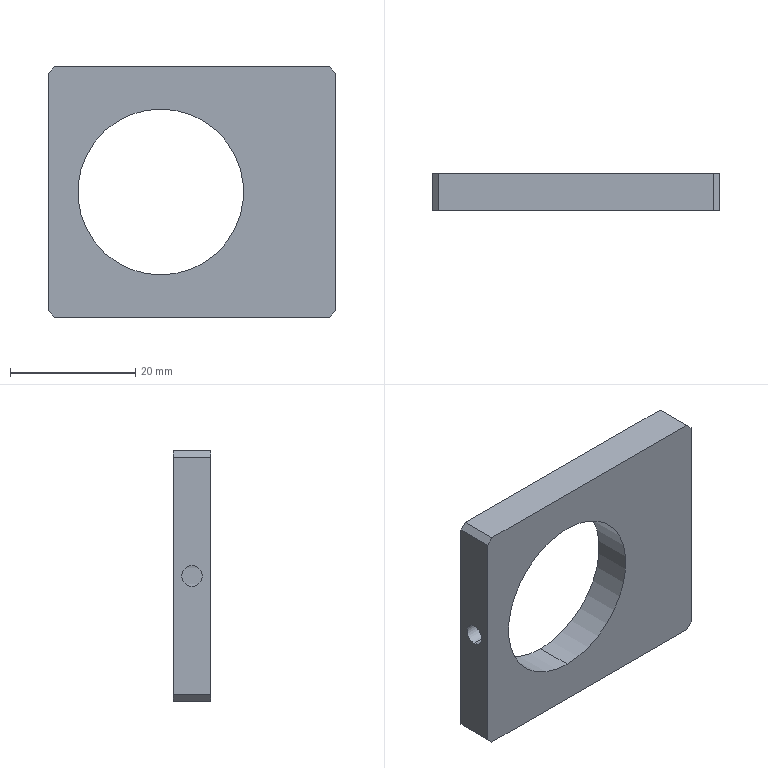Component | SolidWorks | MTCTV2104DJ006-000-0040LimitingPart-1 | 1 solid | 22 faces | box 46 x 6 x 40 mm | volume 7499 mm3 | plane 10 | cylinder 8 | cone 4 | commonest cylinder face diameters 3.3 x6 26.5 x2
build123d program:
from build123d import *

# Parameters (mm, degrees)
SKETCH1_W              = 40
SKETCH1_H              = 46
BOSS_EXTRUDE1_DEPTH    = 6
SKETCH4_R              = 13.25
CUT_EXTRUDE1_DEPTH     = 32.064
M4_TAPPED_HOLE1_REACH  = 52.517
M4_TAPPED_HOLE1_BORE_R = 1.65
M4_TAPPED_HOLE2_D      = 3.3
M4_TAPPED_HOLE2_DEPTH  = 10.1
M4_TAPPED_HOLE2_TIP    = 0.9914
CHAMFER1_SIZE          = 1


with BuildPart() as part:
    # Sketch1 → Boss-Extrude1 (new body)
    with BuildSketch(Plane(origin=(0, 0, 0), x_dir=(0, 0, -1), z_dir=(1, 0, 0))):
        Rectangle(SKETCH1_W, SKETCH1_H)
    extrude(amount=BOSS_EXTRUDE1_DEPTH)

    # Sketch4 → Cut-Extrude1 (cut, through all)
    with BuildSketch(Plane(origin=(6, 0, 0), x_dir=(0, 0, -1), z_dir=(1, 0, 0))):
        with Locations((0, -5)):
            Circle(SKETCH4_R)
    extrude(amount=-CUT_EXTRUDE1_DEPTH, mode=Mode.SUBTRACT)

    # M4 Tapped Hole1 bore → M4 Tapped Hole1 (cut, up to next)
    with BuildSketch(Plane(origin=(0, -23, 0), x_dir=(-1, 0, 0), z_dir=(0, -1, 0)), mode=Mode.PRIVATE) as m4_tapped_hole1_sk1:
        with Locations((-3, 0)):
            Circle(M4_TAPPED_HOLE1_BORE_R)
    m4_tapped_hole1_tool1 = extrude(m4_tapped_hole1_sk1.sketch, amount=-M4_TAPPED_HOLE1_REACH, mode=Mode.PRIVATE) & part.part
    add(m4_tapped_hole1_tool1.solids().sort_by_distance((3, -23, 0))[0], mode=Mode.SUBTRACT)

    # M4 Tapped Hole2
    with Locations(Plane(origin=(0, 23, 0), x_dir=(1, 0, 0), z_dir=(0, 1, 0))):
        with Locations((3, 16), (3, -16)):
            Hole(M4_TAPPED_HOLE2_D / 2, depth=M4_TAPPED_HOLE2_DEPTH)
            with Locations((0, 0, -(M4_TAPPED_HOLE2_DEPTH + M4_TAPPED_HOLE2_TIP / 2))):  # 118° drill point
                Cone(0, M4_TAPPED_HOLE2_D / 2, M4_TAPPED_HOLE2_TIP, mode=Mode.SUBTRACT)

    # Chamfer1
    chamfer1_edges = [part.edges().sort_by_distance(p)[0] for p in [
        (3, -23, -20),
        (3, -23, 20),
        (3, 23, 20),
        (3, 23, -20),
    ]]
    chamfer(chamfer1_edges, length=CHAMFER1_SIZE)


solid = part.part

# Placed as in the assembly
solid = solid.moved(Location((8.798, -27.678, 265.447), (0, 0, -90)))
STEP:
#1=COLOUR_RGB('',0.7922,0.8196,0.9333);
#2=FILL_AREA_STYLE_COLOUR('',#1);
#3=FILL_AREA_STYLE('',(#2));
#4=SURFACE_STYLE_FILL_AREA(#3);
#5=SURFACE_SIDE_STYLE('',(#4));
#6=SURFACE_STYLE_USAGE(.BOTH.,#5);
#7=PRESENTATION_STYLE_ASSIGNMENT((#6));
#8=CARTESIAN_POINT('',(0.8543,-1.208,11.146));
#9=VERTEX_POINT('',#8);
#10=CARTESIAN_POINT('',(0.8543,-1.208,11.016));
#11=VERTEX_POINT('',#10);
#12=CARTESIAN_POINT('',(0.8543,-1.208,11.081));
#13=DIRECTION('',(1.,0.,0.));
#14=DIRECTION('',(0.,0.,-1.));
#15=AXIS2_PLACEMENT_3D('',#12,#13,#14);
#16=CIRCLE('',#15,0.06496);
#17=EDGE_CURVE('',#9,#11,#16,.T.);
#18=ORIENTED_EDGE('',*,*,#17,.F.);
#19=CARTESIAN_POINT('',(1.252,-1.208,11.146));
#20=VERTEX_POINT('',#19);
#21=CARTESIAN_POINT('',(1.252,-1.208,11.146));
#22=DIRECTION('',(1.,0.,0.));
#23=VECTOR('',#22,39.37);
#24=LINE('',#21,#23);
#25=EDGE_CURVE('',#9,#20,#24,.T.);
#26=ORIENTED_EDGE('',*,*,#25,.T.);
#27=CARTESIAN_POINT('',(1.252,-1.208,11.016));
#28=VERTEX_POINT('',#27);
#29=CARTESIAN_POINT('',(1.252,-1.208,11.081));
#30=DIRECTION('',(1.,0.,0.));
#31=DIRECTION('',(0.,0.,-1.));
#32=AXIS2_PLACEMENT_3D('',#29,#30,#31);
#33=CIRCLE('',#32,0.06496);
#34=EDGE_CURVE('',#20,#28,#33,.T.);
#35=ORIENTED_EDGE('',*,*,#34,.T.);
#36=CARTESIAN_POINT('',(1.252,-1.208,11.016));
#37=DIRECTION('',(1.,0.,0.));
#38=VECTOR('',#37,39.37);
#39=LINE('',#36,#38);
#40=EDGE_CURVE('',#11,#28,#39,.T.);
#41=ORIENTED_EDGE('',*,*,#40,.F.);
#42=EDGE_LOOP('',(#18,#26,#35,#41));
#43=FACE_OUTER_BOUND('',#42,.T.);
#44=CARTESIAN_POINT('',(1.252,-1.208,11.081));
#45=DIRECTION('',(1.,0.,0.));
#46=DIRECTION('',(0.,0.,-1.));
#47=AXIS2_PLACEMENT_3D('',#44,#45,#46);
#48=CYLINDRICAL_SURFACE('',#47,0.06496);
#49=ADVANCED_FACE('',(#43),#48,.F.);
#50=CARTESIAN_POINT('',(0.8152,-1.208,11.081));
#51=VERTEX_POINT('',#50);
#52=CARTESIAN_POINT('',(0.8543,-1.208,11.016));
#53=DIRECTION('',(0.515,0.,-0.8572));
#54=VECTOR('',#53,39.37);
#55=LINE('',#52,#54);
#56=EDGE_CURVE('',#51,#11,#55,.T.);
#57=ORIENTED_EDGE('',*,*,#56,.F.);
#58=CARTESIAN_POINT('',(0.8543,-1.208,11.146));
#59=DIRECTION('',(0.515,-0.,0.8572));
#60=VECTOR('',#59,39.37);
#61=LINE('',#58,#60);
#62=EDGE_CURVE('',#51,#9,#61,.T.);
#63=ORIENTED_EDGE('',*,*,#62,.T.);
#64=ORIENTED_EDGE('',*,*,#17,.T.);
#65=EDGE_LOOP('',(#57,#63,#64));
#66=FACE_OUTER_BOUND('',#65,.T.);
#67=CARTESIAN_POINT('',(0.8543,-1.208,11.081));
#68=DIRECTION('',(1.,0.,0.));
#69=DIRECTION('',(0.,0.,-1.));
#70=AXIS2_PLACEMENT_3D('',#67,#68,#69);
#71=CONICAL_SURFACE('',#70,0.06496,1.03);
#72=ADVANCED_FACE('',(#66),#71,.F.);
#73=CARTESIAN_POINT('',(0.8543,-1.208,9.886));
#74=VERTEX_POINT('',#73);
#75=CARTESIAN_POINT('',(0.8543,-1.208,9.756));
#76=VERTEX_POINT('',#75);
#77=CARTESIAN_POINT('',(0.8543,-1.208,9.821));
#78=DIRECTION('',(1.,0.,0.));
#79=DIRECTION('',(0.,0.,-1.));
#80=AXIS2_PLACEMENT_3D('',#77,#78,#79);
#81=CIRCLE('',#80,0.06496);
#82=EDGE_CURVE('',#74,#76,#81,.T.);
#83=ORIENTED_EDGE('',*,*,#82,.F.);
#84=CARTESIAN_POINT('',(1.252,-1.208,9.886));
#85=VERTEX_POINT('',#84);
#86=CARTESIAN_POINT('',(1.252,-1.208,9.886));
#87=DIRECTION('',(1.,0.,0.));
#88=VECTOR('',#87,39.37);
#89=LINE('',#86,#88);
#90=EDGE_CURVE('',#74,#85,#89,.T.);
#91=ORIENTED_EDGE('',*,*,#90,.T.);
#92=CARTESIAN_POINT('',(1.252,-1.208,9.756));
#93=VERTEX_POINT('',#92);
#94=CARTESIAN_POINT('',(1.252,-1.208,9.821));
#95=DIRECTION('',(1.,0.,0.));
#96=DIRECTION('',(0.,0.,-1.));
#97=AXIS2_PLACEMENT_3D('',#94,#95,#96);
#98=CIRCLE('',#97,0.06496);
#99=EDGE_CURVE('',#85,#93,#98,.T.);
#100=ORIENTED_EDGE('',*,*,#99,.T.);
#101=CARTESIAN_POINT('',(1.252,-1.208,9.756));
#102=DIRECTION('',(1.,0.,0.));
#103=VECTOR('',#102,39.37);
#104=LINE('',#101,#103);
#105=EDGE_CURVE('',#76,#93,#104,.T.);
#106=ORIENTED_EDGE('',*,*,#105,.F.);
#107=EDGE_LOOP('',(#83,#91,#100,#106));
#108=FACE_OUTER_BOUND('',#107,.T.);
#109=CARTESIAN_POINT('',(1.252,-1.208,9.821));
#110=DIRECTION('',(1.,0.,0.));
#111=DIRECTION('',(0.,0.,-1.));
#112=AXIS2_PLACEMENT_3D('',#109,#110,#111);
#113=CYLINDRICAL_SURFACE('',#112,0.06496);
#114=ADVANCED_FACE('',(#108),#113,.F.);
#115=CARTESIAN_POINT('',(0.8152,-1.208,9.821));
#116=VERTEX_POINT('',#115);
#117=CARTESIAN_POINT('',(0.8543,-1.208,9.756));
#118=DIRECTION('',(0.515,0.,-0.8572));
#119=VECTOR('',#118,39.37);
#120=LINE('',#117,#119);
#121=EDGE_CURVE('',#116,#76,#120,.T.);
#122=ORIENTED_EDGE('',*,*,#121,.F.);
#123=CARTESIAN_POINT('',(0.8543,-1.208,9.886));
#124=DIRECTION('',(0.515,-0.,0.8572));
#125=VECTOR('',#124,39.37);
#126=LINE('',#123,#125);
#127=EDGE_CURVE('',#116,#74,#126,.T.);
#128=ORIENTED_EDGE('',*,*,#127,.T.);
#129=ORIENTED_EDGE('',*,*,#82,.T.);
#130=EDGE_LOOP('',(#122,#128,#129));
#131=FACE_OUTER_BOUND('',#130,.T.);
#132=CARTESIAN_POINT('',(0.8543,-1.208,9.821));
#133=DIRECTION('',(1.,0.,0.));
#134=DIRECTION('',(0.,0.,-1.));
#135=AXIS2_PLACEMENT_3D('',#132,#133,#134);
#136=CONICAL_SURFACE('',#135,0.06496,1.03);
#137=ADVANCED_FACE('',(#131),#136,.F.);
#138=CARTESIAN_POINT('',(-0.368,-1.208,10.386));
#139=VERTEX_POINT('',#138);
#140=CARTESIAN_POINT('',(-0.368,-1.208,10.516));
#141=VERTEX_POINT('',#140);
#142=CARTESIAN_POINT('',(-0.368,-1.208,10.386));
#143=CARTESIAN_POINT('',(-0.368,-1.216,10.386));
#144=CARTESIAN_POINT('',(-0.3683,-1.225,10.387));
#145=CARTESIAN_POINT('',(-0.369,-1.24,10.394));
#146=CARTESIAN_POINT('',(-0.3695,-1.248,10.399));
#147=CARTESIAN_POINT('',(-0.3703,-1.257,10.408));
#148=CARTESIAN_POINT('',(-0.3706,-1.259,10.411));
#149=CARTESIAN_POINT('',(-0.3711,-1.264,10.418));
#150=CARTESIAN_POINT('',(-0.3713,-1.266,10.422));
#151=CARTESIAN_POINT('',(-0.3717,-1.269,10.43));
#152=CARTESIAN_POINT('',(-0.3719,-1.271,10.434));
#153=CARTESIAN_POINT('',(-0.3721,-1.272,10.442));
#154=CARTESIAN_POINT('',(-0.3721,-1.273,10.446));
#155=CARTESIAN_POINT('',(-0.3721,-1.273,10.455));
#156=CARTESIAN_POINT('',(-0.3721,-1.272,10.459));
#157=CARTESIAN_POINT('',(-0.3719,-1.271,10.467));
#158=CARTESIAN_POINT('',(-0.3717,-1.269,10.472));
#159=CARTESIAN_POINT('',(-0.3713,-1.266,10.479));
#160=CARTESIAN_POINT('',(-0.3711,-1.264,10.483));
#161=CARTESIAN_POINT('',(-0.3706,-1.259,10.49));
#162=CARTESIAN_POINT('',(-0.3703,-1.257,10.494));
#163=CARTESIAN_POINT('',(-0.3696,-1.248,10.503));
#164=CARTESIAN_POINT('',(-0.369,-1.241,10.507));
#165=CARTESIAN_POINT('',(-0.3683,-1.225,10.514));
#166=CARTESIAN_POINT('',(-0.368,-1.216,10.516));
#167=CARTESIAN_POINT('',(-0.368,-1.208,10.516));
#168=B_SPLINE_CURVE_WITH_KNOTS('',3,(#142,#143,#144,#145,#146,#147,#148,#149,#150,#151,#152,#153,#154,#155,#156,#157,#158,#159,#160,#161,#162,#163,#164,#165,#166,#167),.UNSPECIFIED.,.F.,.F.,(4,2,2,2,2,2,2,2,2,2,2,2,4),(0.005164,0.005809,0.006454,0.006777,0.0071,0.007422,0.007745,0.008068,0.00839,0.008713,0.009035,0.009681,0.01033),.UNSPECIFIED.);
#169=EDGE_CURVE('',#139,#141,#168,.T.);
#170=ORIENTED_EDGE('',*,*,#169,.F.);
#171=CARTESIAN_POINT('',(-0.5591,-1.208,10.386));
#172=VERTEX_POINT('',#171);
#173=CARTESIAN_POINT('',(-0.5591,-1.208,10.386));
#174=DIRECTION('',(-1.,-0.,-0.));
#175=VECTOR('',#174,39.37);
#176=LINE('',#173,#175);
#177=EDGE_CURVE('',#139,#172,#176,.T.);
#178=ORIENTED_EDGE('',*,*,#177,.T.);
#179=CARTESIAN_POINT('',(-0.5591,-1.208,10.516));
#180=VERTEX_POINT('',#179);
#181=CARTESIAN_POINT('',(-0.5591,-1.208,10.451));
#182=DIRECTION('',(-1.,-0.,-0.));
#183=DIRECTION('',(0.,0.,1.));
#184=AXIS2_PLACEMENT_3D('',#181,#182,#183);
#185=CIRCLE('',#184,0.06496);
#186=EDGE_CURVE('',#172,#180,#185,.T.);
#187=ORIENTED_EDGE('',*,*,#186,.T.);
#188=CARTESIAN_POINT('',(-0.5591,-1.208,10.516));
#189=DIRECTION('',(-1.,-0.,-0.));
#190=VECTOR('',#189,39.37);
#191=LINE('',#188,#190);
#192=EDGE_CURVE('',#141,#180,#191,.T.);
#193=ORIENTED_EDGE('',*,*,#192,.F.);
#194=EDGE_LOOP('',(#170,#178,#187,#193));
#195=FACE_OUTER_BOUND('',#194,.T.);
#196=CARTESIAN_POINT('',(-0.5591,-1.208,10.451));
#197=DIRECTION('',(-1.,-0.,-0.));
#198=DIRECTION('',(0.,0.,1.));
#199=AXIS2_PLACEMENT_3D('',#196,#197,#198);
#200=CYLINDRICAL_SURFACE('',#199,0.06496);
#201=ADVANCED_FACE('',(#195),#200,.F.);
#202=CARTESIAN_POINT('',(-0.368,-1.208,10.516));
#203=CARTESIAN_POINT('',(-0.368,-1.203,10.516));
#204=CARTESIAN_POINT('',(-0.3681,-1.199,10.515));
#205=CARTESIAN_POINT('',(-0.3683,-1.191,10.514));
#206=CARTESIAN_POINT('',(-0.3685,-1.187,10.512));
#207=CARTESIAN_POINT('',(-0.3688,-1.179,10.509));
#208=CARTESIAN_POINT('',(-0.3691,-1.175,10.507));
#209=CARTESIAN_POINT('',(-0.3695,-1.168,10.502));
#210=CARTESIAN_POINT('',(-0.3698,-1.165,10.5));
#211=CARTESIAN_POINT('',(-0.3706,-1.156,10.491));
#212=CARTESIAN_POINT('',(-0.3711,-1.151,10.483));
#213=CARTESIAN_POINT('',(-0.3719,-1.145,10.468));
#214=CARTESIAN_POINT('',(-0.3721,-1.143,10.459));
#215=CARTESIAN_POINT('',(-0.3721,-1.143,10.446));
#216=CARTESIAN_POINT('',(-0.3721,-1.143,10.442));
#217=CARTESIAN_POINT('',(-0.3719,-1.145,10.434));
#218=CARTESIAN_POINT('',(-0.3717,-1.146,10.43));
#219=CARTESIAN_POINT('',(-0.3713,-1.149,10.422));
#220=CARTESIAN_POINT('',(-0.3711,-1.151,10.418));
#221=CARTESIAN_POINT('',(-0.3706,-1.156,10.411));
#222=CARTESIAN_POINT('',(-0.3703,-1.159,10.408));
#223=CARTESIAN_POINT('',(-0.3698,-1.165,10.402));
#224=CARTESIAN_POINT('',(-0.3695,-1.168,10.399));
#225=CARTESIAN_POINT('',(-0.3691,-1.175,10.394));
#226=CARTESIAN_POINT('',(-0.3688,-1.179,10.392));
#227=CARTESIAN_POINT('',(-0.3685,-1.187,10.389));
#228=CARTESIAN_POINT('',(-0.3683,-1.191,10.388));
#229=CARTESIAN_POINT('',(-0.3681,-1.199,10.386));
#230=CARTESIAN_POINT('',(-0.368,-1.204,10.386));
#231=CARTESIAN_POINT('',(-0.368,-1.208,10.386));
#232=B_SPLINE_CURVE_WITH_KNOTS('',3,(#202,#203,#204,#205,#206,#207,#208,#209,#210,#211,#212,#213,#214,#215,#216,#217,#218,#219,#220,#221,#222,#223,#224,#225,#226,#227,#228,#229,#230,#231),.UNSPECIFIED.,.F.,.F.,(4,2,2,2,2,2,2,2,2,2,2,2,2,2,4),(0.,0.0003227,0.0006455,0.0009682,0.001291,0.001936,0.002582,0.002905,0.003227,0.00355,0.003873,0.004195,0.004518,0.004841,0.005164),.UNSPECIFIED.);
#233=EDGE_CURVE('',#141,#139,#232,.T.);
#234=ORIENTED_EDGE('',*,*,#233,.T.);
#235=ORIENTED_EDGE('',*,*,#169,.T.);
#236=EDGE_LOOP('',(#234,#235));
#237=FACE_BOUND('',#236,.T.);
#238=CARTESIAN_POINT('',(0.1495,-1.326,9.929));
#239=VERTEX_POINT('',#238);
#240=CARTESIAN_POINT('',(0.1495,-1.326,10.972));
#241=VERTEX_POINT('',#240);
#242=CARTESIAN_POINT('',(0.1495,-1.326,10.451));
#243=DIRECTION('',(-0.,1.,0.));
#244=DIRECTION('',(-0.,-0.,1.));
#245=AXIS2_PLACEMENT_3D('',#242,#243,#244);
#246=CIRCLE('',#245,0.5217);
#247=EDGE_CURVE('',#239,#241,#246,.T.);
#248=ORIENTED_EDGE('',*,*,#247,.F.);
#249=CARTESIAN_POINT('',(0.1495,-1.09,9.929));
#250=VERTEX_POINT('',#249);
#251=CARTESIAN_POINT('',(0.1495,-1.326,9.929));
#252=DIRECTION('',(-0.,1.,0.));
#253=VECTOR('',#252,39.37);
#254=LINE('',#251,#253);
#255=EDGE_CURVE('',#239,#250,#254,.T.);
#256=ORIENTED_EDGE('',*,*,#255,.T.);
#257=CARTESIAN_POINT('',(0.1495,-1.09,10.972));
#258=VERTEX_POINT('',#257);
#259=CARTESIAN_POINT('',(0.1495,-1.09,10.451));
#260=DIRECTION('',(-0.,1.,0.));
#261=DIRECTION('',(-0.,-0.,1.));
#262=AXIS2_PLACEMENT_3D('',#259,#260,#261);
#263=CIRCLE('',#262,0.5217);
#264=EDGE_CURVE('',#250,#258,#263,.T.);
#265=ORIENTED_EDGE('',*,*,#264,.T.);
#266=CARTESIAN_POINT('',(0.1495,-1.326,10.972));
#267=DIRECTION('',(-0.,1.,0.));
#268=VECTOR('',#267,39.37);
#269=LINE('',#266,#268);
#270=EDGE_CURVE('',#241,#258,#269,.T.);
#271=ORIENTED_EDGE('',*,*,#270,.F.);
#272=EDGE_LOOP('',(#248,#256,#265,#271));
#273=FACE_OUTER_BOUND('',#272,.T.);
#274=CARTESIAN_POINT('',(0.1495,-1.326,10.451));
#275=DIRECTION('',(-0.,1.,0.));
#276=DIRECTION('',(-0.,-0.,1.));
#277=AXIS2_PLACEMENT_3D('',#274,#275,#276);
#278=CYLINDRICAL_SURFACE('',#277,0.5217);
#279=ADVANCED_FACE('',(#237,#273),#278,.F.);
#280=CARTESIAN_POINT('',(-0.5197,-1.326,11.238));
#281=VERTEX_POINT('',#280);
#282=CARTESIAN_POINT('',(1.213,-1.326,11.238));
#283=VERTEX_POINT('',#282);
#284=CARTESIAN_POINT('',(-0.5591,-1.326,11.238));
#285=DIRECTION('',(1.,0.,0.));
#286=VECTOR('',#285,39.37);
#287=LINE('',#284,#286);
#288=EDGE_CURVE('',#281,#283,#287,.T.);
#289=ORIENTED_EDGE('',*,*,#288,.T.);
#290=CARTESIAN_POINT('',(1.213,-1.09,11.238));
#291=VERTEX_POINT('',#290);
#292=CARTESIAN_POINT('',(1.213,-1.09,11.238));
#293=DIRECTION('',(-0.,1.,0.));
#294=VECTOR('',#293,39.37);
#295=LINE('',#292,#294);
#296=EDGE_CURVE('',#283,#291,#295,.T.);
#297=ORIENTED_EDGE('',*,*,#296,.T.);
#298=CARTESIAN_POINT('',(-0.5197,-1.09,11.238));
#299=VERTEX_POINT('',#298);
#300=CARTESIAN_POINT('',(-0.5591,-1.09,11.238));
#301=DIRECTION('',(1.,0.,0.));
#302=VECTOR('',#301,39.37);
#303=LINE('',#300,#302);
#304=EDGE_CURVE('',#299,#291,#303,.T.);
#305=ORIENTED_EDGE('',*,*,#304,.F.);
#306=CARTESIAN_POINT('',(-0.5197,-1.09,11.238));
#307=DIRECTION('',(0.,-1.,-0.));
#308=VECTOR('',#307,39.37);
#309=LINE('',#306,#308);
#310=EDGE_CURVE('',#299,#281,#309,.T.);
#311=ORIENTED_EDGE('',*,*,#310,.T.);
#312=EDGE_LOOP('',(#289,#297,#305,#311));
#313=FACE_OUTER_BOUND('',#312,.T.);
#314=CARTESIAN_POINT('',(-0.5591,-1.09,11.238));
#315=DIRECTION('',(0.,0.,-1.));
#316=DIRECTION('',(-0.,1.,0.));
#317=AXIS2_PLACEMENT_3D('',#314,#315,#316);
#318=PLANE('',#317);
#319=ADVANCED_FACE('',(#313),#318,.F.);
#320=CARTESIAN_POINT('',(1.252,-1.208,11.081));
#321=DIRECTION('',(1.,0.,0.));
#322=DIRECTION('',(0.,0.,-1.));
#323=AXIS2_PLACEMENT_3D('',#320,#321,#322);
#324=CIRCLE('',#323,0.06496);
#325=EDGE_CURVE('',#28,#20,#324,.T.);
#326=ORIENTED_EDGE('',*,*,#325,.F.);
#327=ORIENTED_EDGE('',*,*,#34,.F.);
#328=EDGE_LOOP('',(#326,#327));
#329=FACE_BOUND('',#328,.T.);
#330=CARTESIAN_POINT('',(1.252,-1.208,9.821));
#331=DIRECTION('',(1.,0.,0.));
#332=DIRECTION('',(0.,0.,-1.));
#333=AXIS2_PLACEMENT_3D('',#330,#331,#332);
#334=CIRCLE('',#333,0.06496);
#335=EDGE_CURVE('',#93,#85,#334,.T.);
#336=ORIENTED_EDGE('',*,*,#335,.F.);
#337=ORIENTED_EDGE('',*,*,#99,.F.);
#338=EDGE_LOOP('',(#336,#337));
#339=FACE_BOUND('',#338,.T.);
#340=CARTESIAN_POINT('',(1.252,-1.09,11.199));
#341=VERTEX_POINT('',#340);
#342=CARTESIAN_POINT('',(1.252,-1.09,9.703));
#343=VERTEX_POINT('',#342);
#344=CARTESIAN_POINT('',(1.252,-1.09,9.663));
#345=DIRECTION('',(0.,0.,-1.));
#346=VECTOR('',#345,39.37);
#347=LINE('',#344,#346);
#348=EDGE_CURVE('',#341,#343,#347,.T.);
#349=ORIENTED_EDGE('',*,*,#348,.F.);
#350=CARTESIAN_POINT('',(1.252,-1.326,11.199));
#351=VERTEX_POINT('',#350);
#352=CARTESIAN_POINT('',(1.252,-1.09,11.199));
#353=DIRECTION('',(0.,-1.,-0.));
#354=VECTOR('',#353,39.37);
#355=LINE('',#352,#354);
#356=EDGE_CURVE('',#341,#351,#355,.T.);
#357=ORIENTED_EDGE('',*,*,#356,.T.);
#358=CARTESIAN_POINT('',(1.252,-1.326,9.703));
#359=VERTEX_POINT('',#358);
#360=CARTESIAN_POINT('',(1.252,-1.326,9.663));
#361=DIRECTION('',(0.,0.,-1.));
#362=VECTOR('',#361,39.37);
#363=LINE('',#360,#362);
#364=EDGE_CURVE('',#351,#359,#363,.T.);
#365=ORIENTED_EDGE('',*,*,#364,.T.);
#366=CARTESIAN_POINT('',(1.252,-1.09,9.703));
#367=DIRECTION('',(-0.,1.,0.));
#368=VECTOR('',#367,39.37);
#369=LINE('',#366,#368);
#370=EDGE_CURVE('',#359,#343,#369,.T.);
#371=ORIENTED_EDGE('',*,*,#370,.T.);
#372=EDGE_LOOP('',(#349,#357,#365,#371));
#373=FACE_OUTER_BOUND('',#372,.T.);
#374=CARTESIAN_POINT('',(1.252,-1.09,9.663));
#375=DIRECTION('',(-1.,-0.,-0.));
#376=DIRECTION('',(-0.,-0.,1.));
#377=AXIS2_PLACEMENT_3D('',#374,#375,#376);
#378=PLANE('',#377);
#379=ADVANCED_FACE('',(#329,#339,#373),#378,.F.);
#380=CARTESIAN_POINT('',(1.213,-1.09,9.663));
#381=VERTEX_POINT('',#380);
#382=CARTESIAN_POINT('',(-0.5197,-1.09,9.663));
#383=VERTEX_POINT('',#382);
#384=CARTESIAN_POINT('',(-0.5591,-1.09,9.663));
#385=DIRECTION('',(-1.,-0.,-0.));
#386=VECTOR('',#385,39.37);
#387=LINE('',#384,#386);
#388=EDGE_CURVE('',#381,#383,#387,.T.);
#389=ORIENTED_EDGE('',*,*,#388,.F.);
#390=CARTESIAN_POINT('',(1.213,-1.326,9.663));
#391=VERTEX_POINT('',#390);
#392=CARTESIAN_POINT('',(1.213,-1.09,9.663));
#393=DIRECTION('',(0.,-1.,-0.));
#394=VECTOR('',#393,39.37);
#395=LINE('',#392,#394);
#396=EDGE_CURVE('',#381,#391,#395,.T.);
#397=ORIENTED_EDGE('',*,*,#396,.T.);
#398=CARTESIAN_POINT('',(-0.5197,-1.326,9.663));
#399=VERTEX_POINT('',#398);
#400=CARTESIAN_POINT('',(-0.5591,-1.326,9.663));
#401=DIRECTION('',(-1.,-0.,-0.));
#402=VECTOR('',#401,39.37);
#403=LINE('',#400,#402);
#404=EDGE_CURVE('',#391,#399,#403,.T.);
#405=ORIENTED_EDGE('',*,*,#404,.T.);
#406=CARTESIAN_POINT('',(-0.5197,-1.09,9.663));
#407=DIRECTION('',(-0.,1.,0.));
#408=VECTOR('',#407,39.37);
#409=LINE('',#406,#408);
#410=EDGE_CURVE('',#399,#383,#409,.T.);
#411=ORIENTED_EDGE('',*,*,#410,.T.);
#412=EDGE_LOOP('',(#389,#397,#405,#411));
#413=FACE_OUTER_BOUND('',#412,.T.);
#414=CARTESIAN_POINT('',(-0.5591,-1.09,9.663));
#415=DIRECTION('',(-0.,-0.,1.));
#416=DIRECTION('',(0.,-1.,-0.));
#417=AXIS2_PLACEMENT_3D('',#414,#415,#416);
#418=PLANE('',#417);
#419=ADVANCED_FACE('',(#413),#418,.F.);
#420=CARTESIAN_POINT('',(-0.5591,-1.208,10.451));
#421=DIRECTION('',(-1.,-0.,-0.));
#422=DIRECTION('',(0.,0.,1.));
#423=AXIS2_PLACEMENT_3D('',#420,#421,#422);
#424=CIRCLE('',#423,0.06496);
#425=EDGE_CURVE('',#180,#172,#424,.T.);
#426=ORIENTED_EDGE('',*,*,#425,.F.);
#427=ORIENTED_EDGE('',*,*,#186,.F.);
#428=EDGE_LOOP('',(#426,#427));
#429=FACE_BOUND('',#428,.T.);
#430=CARTESIAN_POINT('',(-0.5591,-1.09,9.703));
#431=VERTEX_POINT('',#430);
#432=CARTESIAN_POINT('',(-0.5591,-1.09,11.199));
#433=VERTEX_POINT('',#432);
#434=CARTESIAN_POINT('',(-0.5591,-1.09,9.663));
#435=DIRECTION('',(-0.,-0.,1.));
#436=VECTOR('',#435,39.37);
#437=LINE('',#434,#436);
#438=EDGE_CURVE('',#431,#433,#437,.T.);
#439=ORIENTED_EDGE('',*,*,#438,.F.);
#440=CARTESIAN_POINT('',(-0.5591,-1.326,9.703));
#441=VERTEX_POINT('',#440);
#442=CARTESIAN_POINT('',(-0.5591,-1.09,9.703));
#443=DIRECTION('',(0.,-1.,-0.));
#444=VECTOR('',#443,39.37);
#445=LINE('',#442,#444);
#446=EDGE_CURVE('',#431,#441,#445,.T.);
#447=ORIENTED_EDGE('',*,*,#446,.T.);
#448=CARTESIAN_POINT('',(-0.5591,-1.326,11.199));
#449=VERTEX_POINT('',#448);
#450=CARTESIAN_POINT('',(-0.5591,-1.326,9.663));
#451=DIRECTION('',(-0.,-0.,1.));
#452=VECTOR('',#451,39.37);
#453=LINE('',#450,#452);
#454=EDGE_CURVE('',#441,#449,#453,.T.);
#455=ORIENTED_EDGE('',*,*,#454,.T.);
#456=CARTESIAN_POINT('',(-0.5591,-1.09,11.199));
#457=DIRECTION('',(-0.,1.,0.));
#458=VECTOR('',#457,39.37);
#459=LINE('',#456,#458);
#460=EDGE_CURVE('',#449,#433,#459,.T.);
#461=ORIENTED_EDGE('',*,*,#460,.T.);
#462=EDGE_LOOP('',(#439,#447,#455,#461));
#463=FACE_OUTER_BOUND('',#462,.T.);
#464=CARTESIAN_POINT('',(-0.5591,-1.09,9.663));
#465=DIRECTION('',(1.,0.,0.));
#466=DIRECTION('',(0.,0.,-1.));
#467=AXIS2_PLACEMENT_3D('',#464,#465,#466);
#468=PLANE('',#467);
#469=ADVANCED_FACE('',(#429,#463),#468,.F.);
#470=CARTESIAN_POINT('',(0.1495,-1.09,10.451));
#471=DIRECTION('',(-0.,1.,0.));
#472=DIRECTION('',(-0.,-0.,1.));
#473=AXIS2_PLACEMENT_3D('',#470,#471,#472);
#474=CIRCLE('',#473,0.5217);
#475=EDGE_CURVE('',#258,#250,#474,.T.);
#476=ORIENTED_EDGE('',*,*,#475,.F.);
#477=ORIENTED_EDGE('',*,*,#264,.F.);
#478=EDGE_LOOP('',(#476,#477));
#479=FACE_BOUND('',#478,.T.);
#480=ORIENTED_EDGE('',*,*,#304,.T.);
#481=CARTESIAN_POINT('',(1.252,-1.09,11.199));
#482=DIRECTION('',(0.7071,0.,-0.7071));
#483=VECTOR('',#482,39.37);
#484=LINE('',#481,#483);
#485=EDGE_CURVE('',#291,#341,#484,.T.);
#486=ORIENTED_EDGE('',*,*,#485,.T.);
#487=ORIENTED_EDGE('',*,*,#348,.T.);
#488=CARTESIAN_POINT('',(1.213,-1.09,9.663));
#489=DIRECTION('',(-0.7071,0.,-0.7071));
#490=VECTOR('',#489,39.37);
#491=LINE('',#488,#490);
#492=EDGE_CURVE('',#343,#381,#491,.T.);
#493=ORIENTED_EDGE('',*,*,#492,.T.);
#494=ORIENTED_EDGE('',*,*,#388,.T.);
#495=CARTESIAN_POINT('',(-0.5591,-1.09,9.703));
#496=DIRECTION('',(-0.7071,-0.,0.7071));
#497=VECTOR('',#496,39.37);
#498=LINE('',#495,#497);
#499=EDGE_CURVE('',#383,#431,#498,.T.);
#500=ORIENTED_EDGE('',*,*,#499,.T.);
#501=ORIENTED_EDGE('',*,*,#438,.T.);
#502=CARTESIAN_POINT('',(-0.5197,-1.09,11.238));
#503=DIRECTION('',(0.7071,-0.,0.7071));
#504=VECTOR('',#503,39.37);
#505=LINE('',#502,#504);
#506=EDGE_CURVE('',#433,#299,#505,.T.);
#507=ORIENTED_EDGE('',*,*,#506,.T.);
#508=EDGE_LOOP('',(#480,#486,#487,#493,#494,#500,#501,#507));
#509=FACE_OUTER_BOUND('',#508,.T.);
#510=CARTESIAN_POINT('',(0.3464,-1.09,10.451));
#511=DIRECTION('',(0.,-1.,-0.));
#512=DIRECTION('',(0.,0.,-1.));
#513=AXIS2_PLACEMENT_3D('',#510,#511,#512);
#514=PLANE('',#513);
#515=ADVANCED_FACE('',(#479,#509),#514,.F.);
#516=CARTESIAN_POINT('',(0.1495,-1.326,10.451));
#517=DIRECTION('',(-0.,1.,0.));
#518=DIRECTION('',(-0.,-0.,1.));
#519=AXIS2_PLACEMENT_3D('',#516,#517,#518);
#520=CIRCLE('',#519,0.5217);
#521=EDGE_CURVE('',#241,#239,#520,.T.);
#522=ORIENTED_EDGE('',*,*,#521,.T.);
#523=ORIENTED_EDGE('',*,*,#247,.T.);
#524=EDGE_LOOP('',(#522,#523));
#525=FACE_BOUND('',#524,.T.);
#526=ORIENTED_EDGE('',*,*,#364,.F.);
#527=CARTESIAN_POINT('',(1.173,-1.326,11.277));
#528=DIRECTION('',(-0.7071,-0.,0.7071));
#529=VECTOR('',#528,39.37);
#530=LINE('',#527,#529);
#531=EDGE_CURVE('',#351,#283,#530,.T.);
#532=ORIENTED_EDGE('',*,*,#531,.T.);
#533=ORIENTED_EDGE('',*,*,#288,.F.);
#534=CARTESIAN_POINT('',(-0.4804,-1.326,11.277));
#535=DIRECTION('',(-0.7071,0.,-0.7071));
#536=VECTOR('',#535,39.37);
#537=LINE('',#534,#536);
#538=EDGE_CURVE('',#281,#449,#537,.T.);
#539=ORIENTED_EDGE('',*,*,#538,.T.);
#540=ORIENTED_EDGE('',*,*,#454,.F.);
#541=CARTESIAN_POINT('',(-0.4804,-1.326,9.624));
#542=DIRECTION('',(0.7071,0.,-0.7071));
#543=VECTOR('',#542,39.37);
#544=LINE('',#541,#543);
#545=EDGE_CURVE('',#441,#399,#544,.T.);
#546=ORIENTED_EDGE('',*,*,#545,.T.);
#547=ORIENTED_EDGE('',*,*,#404,.F.);
#548=CARTESIAN_POINT('',(1.173,-1.326,9.624));
#549=DIRECTION('',(0.7071,-0.,0.7071));
#550=VECTOR('',#549,39.37);
#551=LINE('',#548,#550);
#552=EDGE_CURVE('',#391,#359,#551,.T.);
#553=ORIENTED_EDGE('',*,*,#552,.T.);
#554=EDGE_LOOP('',(#526,#532,#533,#539,#540,#546,#547,#553));
#555=FACE_OUTER_BOUND('',#554,.T.);
#556=CARTESIAN_POINT('',(0.3464,-1.326,10.451));
#557=DIRECTION('',(0.,-1.,-0.));
#558=DIRECTION('',(0.,0.,-1.));
#559=AXIS2_PLACEMENT_3D('',#556,#557,#558);
#560=PLANE('',#559);
#561=ADVANCED_FACE('',(#525,#555),#560,.T.);
#562=ORIENTED_EDGE('',*,*,#255,.F.);
#563=ORIENTED_EDGE('',*,*,#521,.F.);
#564=ORIENTED_EDGE('',*,*,#270,.T.);
#565=ORIENTED_EDGE('',*,*,#475,.T.);
#566=EDGE_LOOP('',(#562,#563,#564,#565));
#567=FACE_OUTER_BOUND('',#566,.T.);
#568=CARTESIAN_POINT('',(0.1495,-1.326,10.451));
#569=DIRECTION('',(-0.,1.,0.));
#570=DIRECTION('',(-0.,-0.,1.));
#571=AXIS2_PLACEMENT_3D('',#568,#569,#570);
#572=CYLINDRICAL_SURFACE('',#571,0.5217);
#573=ADVANCED_FACE('',(#567),#572,.F.);
#574=ORIENTED_EDGE('',*,*,#177,.F.);
#575=ORIENTED_EDGE('',*,*,#233,.F.);
#576=ORIENTED_EDGE('',*,*,#192,.T.);
#577=ORIENTED_EDGE('',*,*,#425,.T.);
#578=EDGE_LOOP('',(#574,#575,#576,#577));
#579=FACE_OUTER_BOUND('',#578,.T.);
#580=CARTESIAN_POINT('',(-0.5591,-1.208,10.451));
#581=DIRECTION('',(-1.,-0.,-0.));
#582=DIRECTION('',(0.,0.,1.));
#583=AXIS2_PLACEMENT_3D('',#580,#581,#582);
#584=CYLINDRICAL_SURFACE('',#583,0.06496);
#585=ADVANCED_FACE('',(#579),#584,.F.);
#586=ORIENTED_EDGE('',*,*,#127,.F.);
#587=ORIENTED_EDGE('',*,*,#121,.T.);
#588=CARTESIAN_POINT('',(0.8543,-1.208,9.821));
#589=DIRECTION('',(1.,0.,0.));
#590=DIRECTION('',(0.,0.,-1.));
#591=AXIS2_PLACEMENT_3D('',#588,#589,#590);
#592=CIRCLE('',#591,0.06496);
#593=EDGE_CURVE('',#76,#74,#592,.T.);
#594=ORIENTED_EDGE('',*,*,#593,.T.);
#595=EDGE_LOOP('',(#586,#587,#594));
#596=FACE_OUTER_BOUND('',#595,.T.);
#597=CARTESIAN_POINT('',(0.8543,-1.208,9.821));
#598=DIRECTION('',(1.,0.,0.));
#599=DIRECTION('',(0.,0.,-1.));
#600=AXIS2_PLACEMENT_3D('',#597,#598,#599);
#601=CONICAL_SURFACE('',#600,0.06496,1.03);
#602=ADVANCED_FACE('',(#596),#601,.F.);
#603=ORIENTED_EDGE('',*,*,#90,.F.);
#604=ORIENTED_EDGE('',*,*,#593,.F.);
#605=ORIENTED_EDGE('',*,*,#105,.T.);
#606=ORIENTED_EDGE('',*,*,#335,.T.);
#607=EDGE_LOOP('',(#603,#604,#605,#606));
#608=FACE_OUTER_BOUND('',#607,.T.);
#609=CARTESIAN_POINT('',(1.252,-1.208,9.821));
#610=DIRECTION('',(1.,0.,0.));
#611=DIRECTION('',(0.,0.,-1.));
#612=AXIS2_PLACEMENT_3D('',#609,#610,#611);
#613=CYLINDRICAL_SURFACE('',#612,0.06496);
#614=ADVANCED_FACE('',(#608),#613,.F.);
#615=ORIENTED_EDGE('',*,*,#62,.F.);
#616=ORIENTED_EDGE('',*,*,#56,.T.);
#617=CARTESIAN_POINT('',(0.8543,-1.208,11.081));
#618=DIRECTION('',(1.,0.,0.));
#619=DIRECTION('',(0.,0.,-1.));
#620=AXIS2_PLACEMENT_3D('',#617,#618,#619);
#621=CIRCLE('',#620,0.06496);
#622=EDGE_CURVE('',#11,#9,#621,.T.);
#623=ORIENTED_EDGE('',*,*,#622,.T.);
#624=EDGE_LOOP('',(#615,#616,#623));
#625=FACE_OUTER_BOUND('',#624,.T.);
#626=CARTESIAN_POINT('',(0.8543,-1.208,11.081));
#627=DIRECTION('',(1.,0.,0.));
#628=DIRECTION('',(0.,0.,-1.));
#629=AXIS2_PLACEMENT_3D('',#626,#627,#628);
#630=CONICAL_SURFACE('',#629,0.06496,1.03);
#631=ADVANCED_FACE('',(#625),#630,.F.);
#632=ORIENTED_EDGE('',*,*,#25,.F.);
#633=ORIENTED_EDGE('',*,*,#622,.F.);
#634=ORIENTED_EDGE('',*,*,#40,.T.);
#635=ORIENTED_EDGE('',*,*,#325,.T.);
#636=EDGE_LOOP('',(#632,#633,#634,#635));
#637=FACE_OUTER_BOUND('',#636,.T.);
#638=CARTESIAN_POINT('',(1.252,-1.208,11.081));
#639=DIRECTION('',(1.,0.,0.));
#640=DIRECTION('',(0.,0.,-1.));
#641=AXIS2_PLACEMENT_3D('',#638,#639,#640);
#642=CYLINDRICAL_SURFACE('',#641,0.06496);
#643=ADVANCED_FACE('',(#637),#642,.F.);
#644=ORIENTED_EDGE('',*,*,#485,.F.);
#645=ORIENTED_EDGE('',*,*,#296,.F.);
#646=ORIENTED_EDGE('',*,*,#531,.F.);
#647=ORIENTED_EDGE('',*,*,#356,.F.);
#648=EDGE_LOOP('',(#644,#645,#646,#647));
#649=FACE_OUTER_BOUND('',#648,.T.);
#650=CARTESIAN_POINT('',(1.252,-1.09,11.199));
#651=DIRECTION('',(-0.7071,0.,-0.7071));
#652=DIRECTION('',(0.,-1.,-0.));
#653=AXIS2_PLACEMENT_3D('',#650,#651,#652);
#654=PLANE('',#653);
#655=ADVANCED_FACE('',(#649),#654,.F.);
#656=ORIENTED_EDGE('',*,*,#492,.F.);
#657=ORIENTED_EDGE('',*,*,#370,.F.);
#658=ORIENTED_EDGE('',*,*,#552,.F.);
#659=ORIENTED_EDGE('',*,*,#396,.F.);
#660=EDGE_LOOP('',(#656,#657,#658,#659));
#661=FACE_OUTER_BOUND('',#660,.T.);
#662=CARTESIAN_POINT('',(1.213,-1.09,9.663));
#663=DIRECTION('',(-0.7071,-0.,0.7071));
#664=DIRECTION('',(0.,-1.,-0.));
#665=AXIS2_PLACEMENT_3D('',#662,#663,#664);
#666=PLANE('',#665);
#667=ADVANCED_FACE('',(#661),#666,.F.);
#668=ORIENTED_EDGE('',*,*,#499,.F.);
#669=ORIENTED_EDGE('',*,*,#410,.F.);
#670=ORIENTED_EDGE('',*,*,#545,.F.);
#671=ORIENTED_EDGE('',*,*,#446,.F.);
#672=EDGE_LOOP('',(#668,#669,#670,#671));
#673=FACE_OUTER_BOUND('',#672,.T.);
#674=CARTESIAN_POINT('',(-0.5591,-1.09,9.703));
#675=DIRECTION('',(0.7071,-0.,0.7071));
#676=DIRECTION('',(0.,-1.,-0.));
#677=AXIS2_PLACEMENT_3D('',#674,#675,#676);
#678=PLANE('',#677);
#679=ADVANCED_FACE('',(#673),#678,.F.);
#680=ORIENTED_EDGE('',*,*,#506,.F.);
#681=ORIENTED_EDGE('',*,*,#460,.F.);
#682=ORIENTED_EDGE('',*,*,#538,.F.);
#683=ORIENTED_EDGE('',*,*,#310,.F.);
#684=EDGE_LOOP('',(#680,#681,#682,#683));
#685=FACE_OUTER_BOUND('',#684,.T.);
#686=CARTESIAN_POINT('',(-0.5197,-1.09,11.238));
#687=DIRECTION('',(0.7071,0.,-0.7071));
#688=DIRECTION('',(0.,-1.,-0.));
#689=AXIS2_PLACEMENT_3D('',#686,#687,#688);
#690=PLANE('',#689);
#691=ADVANCED_FACE('',(#685),#690,.F.);
#692=CLOSED_SHELL('',(#49,#72,#114,#137,#201,#279,#319,#379,#419,#469,#515,#561,#573,#585,#602,#614,#631,#643,#655,#667,#679,#691));
#693=MANIFOLD_SOLID_BREP('',#692);
#694=STYLED_ITEM('',(#7),#693);
#695=(LENGTH_UNIT()NAMED_UNIT(*)SI_UNIT($,.METRE.));
#696=LENGTH_MEASURE_WITH_UNIT(LENGTH_MEASURE(0.0254),#695);
#697=DIMENSIONAL_EXPONENTS(1.,0.,0.,0.,0.,0.,0.);
#698=(CONVERSION_BASED_UNIT('',#696)LENGTH_UNIT()NAMED_UNIT(#697));
#699=UNCERTAINTY_MEASURE_WITH_UNIT(LENGTH_MEASURE(0.00001),#698,'','');
#700=(NAMED_UNIT(*)PLANE_ANGLE_UNIT()SI_UNIT($,.RADIAN.));
#701=(NAMED_UNIT(*)SI_UNIT($,.STERADIAN.)SOLID_ANGLE_UNIT());
#702=(GEOMETRIC_REPRESENTATION_CONTEXT(3)GLOBAL_UNCERTAINTY_ASSIGNED_CONTEXT((#699))GLOBAL_UNIT_ASSIGNED_CONTEXT((#698,#700,#701))REPRESENTATION_CONTEXT('',''));
#703=MECHANICAL_DESIGN_GEOMETRIC_PRESENTATION_REPRESENTATION('',(#694),#702);
#704=CARTESIAN_POINT('',(0.,0.,0.));
#705=DIRECTION('',(0.,0.,1.));
#706=DIRECTION('',(1.,0.,0.));
#707=AXIS2_PLACEMENT_3D('',#704,#705,#706);
#708=(LENGTH_UNIT()NAMED_UNIT(*)SI_UNIT($,.METRE.));
#709=LENGTH_MEASURE_WITH_UNIT(LENGTH_MEASURE(0.0254),#708);
#710=DIMENSIONAL_EXPONENTS(1.,0.,0.,0.,0.,0.,0.);
#711=(CONVERSION_BASED_UNIT('',#709)LENGTH_UNIT()NAMED_UNIT(#710));
#712=UNCERTAINTY_MEASURE_WITH_UNIT(LENGTH_MEASURE(0.00001),#711,'','');
#713=(NAMED_UNIT(*)PLANE_ANGLE_UNIT()SI_UNIT($,.RADIAN.));
#714=(NAMED_UNIT(*)SI_UNIT($,.STERADIAN.)SOLID_ANGLE_UNIT());
#715=(GEOMETRIC_REPRESENTATION_CONTEXT(3)GLOBAL_UNCERTAINTY_ASSIGNED_CONTEXT((#712))GLOBAL_UNIT_ASSIGNED_CONTEXT((#711,#713,#714))REPRESENTATION_CONTEXT('',''));
#716=ADVANCED_BREP_SHAPE_REPRESENTATION('',(#693,#707),#715);
#717=PRESENTATION_LAYER_ASSIGNMENT('','',(#694));